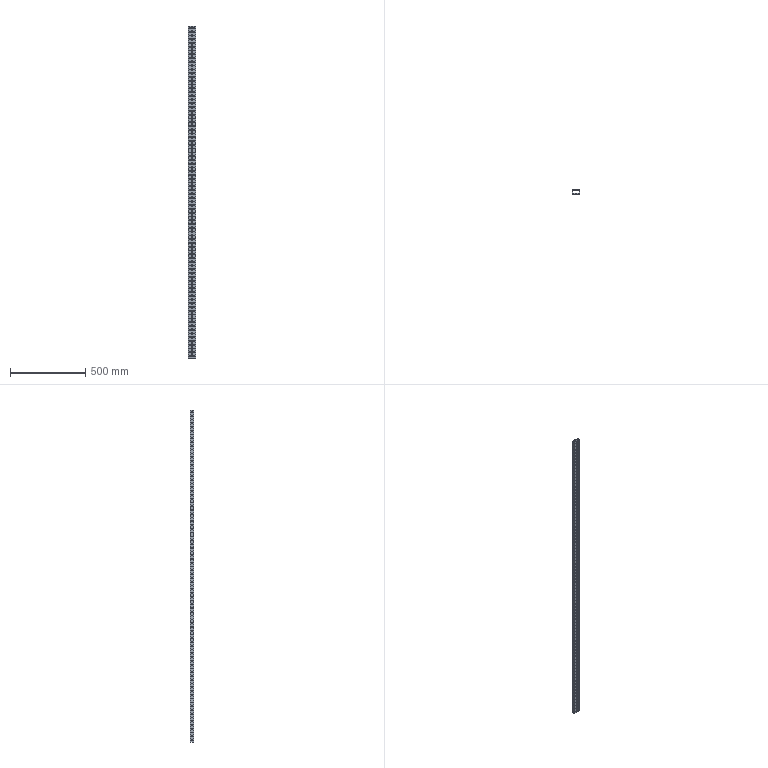Component | SolidWorks | FrontPost-1 | 1 solid | 1094 faces | volume 525882 mm3 | plane 558 | cylinder 536 | commonest cylinder face diameters 5 x528 6 x4 2 x4 | material Plain Carbon Steel